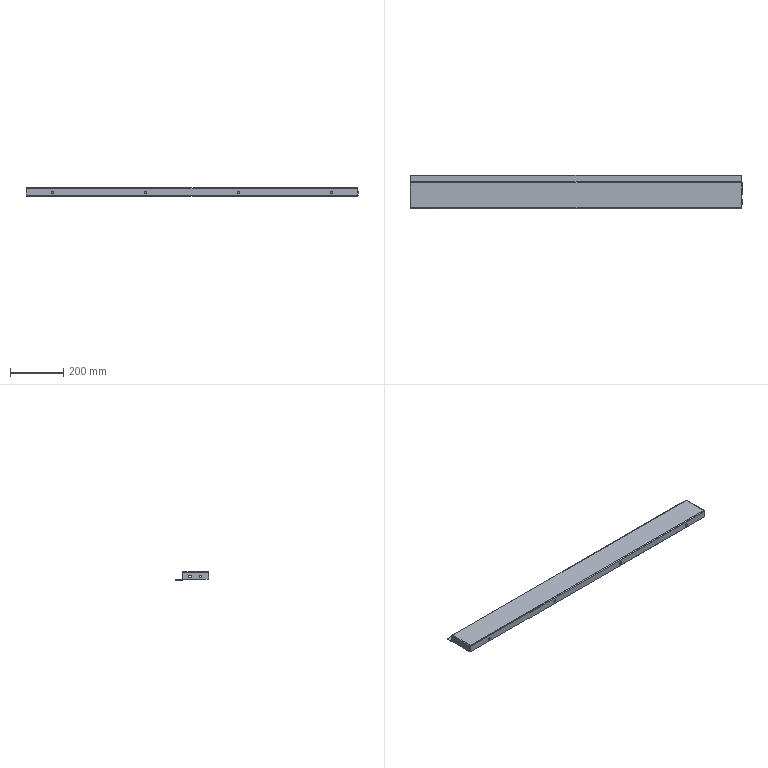Component | SolidWorks | 24BaseFrontSidePlateI-1 | 1 solid | 62 faces | volume 453694 mm3 | plane 28 | cylinder 26 | spline 8 | commonest cylinder face diameters 10 x16 2 x5 6 x5